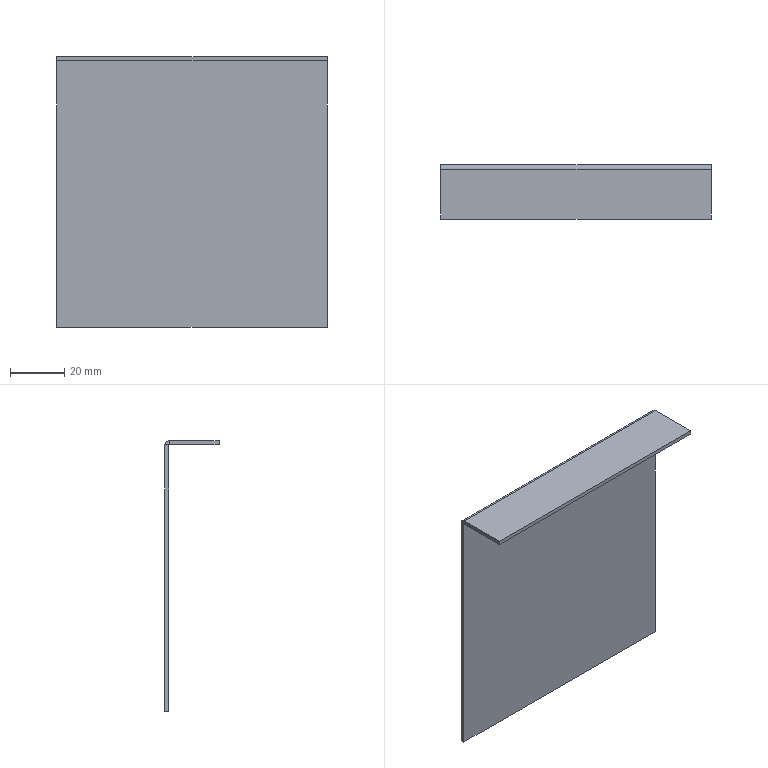Component | SolidWorks | WeldmentDrawing-1_CircuitBreakerBracket-1 | 1 solid | 14 faces | box 100 x 20 x 100 mm | volume 17720 mm3 | plane 12 | cylinder 2 | commonest cylinder face diameters 3.2 x1 0.2 x1
STEP:
#1=COLOUR_RGB('',0.7922,0.8196,0.9333);
#2=FILL_AREA_STYLE_COLOUR('',#1);
#3=FILL_AREA_STYLE('',(#2));
#4=SURFACE_STYLE_FILL_AREA(#3);
#5=SURFACE_SIDE_STYLE('',(#4));
#6=SURFACE_STYLE_USAGE(.BOTH.,#5);
#7=PRESENTATION_STYLE_ASSIGNMENT((#6));
#8=CARTESIAN_POINT('',(1.698,-7.825,-6.929));
#9=VERTEX_POINT('',#8);
#10=CARTESIAN_POINT('',(1.698,-7.825,-3.055));
#11=VERTEX_POINT('',#10);
#12=CARTESIAN_POINT('',(1.698,-7.825,-6.929));
#13=DIRECTION('',(-0.,-0.,1.));
#14=VECTOR('',#13,39.37);
#15=LINE('',#12,#14);
#16=EDGE_CURVE('',#9,#11,#15,.T.);
#17=ORIENTED_EDGE('',*,*,#16,.T.);
#18=CARTESIAN_POINT('',(1.698,-7.766,-3.055));
#19=VERTEX_POINT('',#18);
#20=CARTESIAN_POINT('',(1.698,-7.825,-3.055));
#21=DIRECTION('',(0.,1.,0.));
#22=VECTOR('',#21,39.37);
#23=LINE('',#20,#22);
#24=EDGE_CURVE('',#11,#19,#23,.T.);
#25=ORIENTED_EDGE('',*,*,#24,.T.);
#26=CARTESIAN_POINT('',(1.698,-7.766,-6.929));
#27=VERTEX_POINT('',#26);
#28=CARTESIAN_POINT('',(1.698,-7.766,-6.929));
#29=DIRECTION('',(-0.,-0.,1.));
#30=VECTOR('',#29,39.37);
#31=LINE('',#28,#30);
#32=EDGE_CURVE('',#27,#19,#31,.T.);
#33=ORIENTED_EDGE('',*,*,#32,.F.);
#34=CARTESIAN_POINT('',(1.698,-7.825,-6.929));
#35=DIRECTION('',(0.,1.,0.));
#36=VECTOR('',#35,39.37);
#37=LINE('',#34,#36);
#38=EDGE_CURVE('',#9,#27,#37,.T.);
#39=ORIENTED_EDGE('',*,*,#38,.F.);
#40=EDGE_LOOP('',(#17,#25,#33,#39));
#41=FACE_OUTER_BOUND('',#40,.T.);
#42=CARTESIAN_POINT('',(1.698,-7.825,-6.929));
#43=DIRECTION('',(-1.,-0.,-0.));
#44=DIRECTION('',(-0.,-0.,1.));
#45=AXIS2_PLACEMENT_3D('',#42,#43,#44);
#46=PLANE('',#45);
#47=ADVANCED_FACE('',(#41),#46,.T.);
#48=CARTESIAN_POINT('',(5.635,-7.825,-3.055));
#49=VERTEX_POINT('',#48);
#50=CARTESIAN_POINT('',(5.635,-7.825,-6.929));
#51=VERTEX_POINT('',#50);
#52=CARTESIAN_POINT('',(5.635,-7.825,-6.929));
#53=DIRECTION('',(0.,0.,-1.));
#54=VECTOR('',#53,39.37);
#55=LINE('',#52,#54);
#56=EDGE_CURVE('',#49,#51,#55,.T.);
#57=ORIENTED_EDGE('',*,*,#56,.F.);
#58=CARTESIAN_POINT('',(1.698,-7.825,-3.055));
#59=DIRECTION('',(1.,0.,0.));
#60=VECTOR('',#59,39.37);
#61=LINE('',#58,#60);
#62=EDGE_CURVE('',#11,#49,#61,.T.);
#63=ORIENTED_EDGE('',*,*,#62,.F.);
#64=ORIENTED_EDGE('',*,*,#16,.F.);
#65=CARTESIAN_POINT('',(5.635,-7.825,-6.929));
#66=DIRECTION('',(-1.,0.,-0.));
#67=VECTOR('',#66,39.37);
#68=LINE('',#65,#67);
#69=EDGE_CURVE('',#51,#9,#68,.T.);
#70=ORIENTED_EDGE('',*,*,#69,.F.);
#71=EDGE_LOOP('',(#57,#63,#64,#70));
#72=FACE_OUTER_BOUND('',#71,.T.);
#73=CARTESIAN_POINT('',(3.673,-7.825,-5.041));
#74=DIRECTION('',(-0.,-1.,-0.));
#75=DIRECTION('',(-0.,-0.,1.));
#76=AXIS2_PLACEMENT_3D('',#73,#74,#75);
#77=PLANE('',#76);
#78=ADVANCED_FACE('',(#72),#77,.T.);
#79=CARTESIAN_POINT('',(5.635,-7.766,-3.055));
#80=VERTEX_POINT('',#79);
#81=CARTESIAN_POINT('',(1.698,-7.766,-3.055));
#82=DIRECTION('',(1.,0.,0.));
#83=VECTOR('',#82,39.37);
#84=LINE('',#81,#83);
#85=EDGE_CURVE('',#19,#80,#84,.T.);
#86=ORIENTED_EDGE('',*,*,#85,.T.);
#87=CARTESIAN_POINT('',(5.635,-7.766,-6.929));
#88=VERTEX_POINT('',#87);
#89=CARTESIAN_POINT('',(5.635,-7.766,-6.929));
#90=DIRECTION('',(0.,0.,-1.));
#91=VECTOR('',#90,39.37);
#92=LINE('',#89,#91);
#93=EDGE_CURVE('',#80,#88,#92,.T.);
#94=ORIENTED_EDGE('',*,*,#93,.T.);
#95=CARTESIAN_POINT('',(5.635,-7.766,-6.929));
#96=DIRECTION('',(-1.,0.,-0.));
#97=VECTOR('',#96,39.37);
#98=LINE('',#95,#97);
#99=EDGE_CURVE('',#88,#27,#98,.T.);
#100=ORIENTED_EDGE('',*,*,#99,.T.);
#101=ORIENTED_EDGE('',*,*,#32,.T.);
#102=EDGE_LOOP('',(#86,#94,#100,#101));
#103=FACE_OUTER_BOUND('',#102,.T.);
#104=CARTESIAN_POINT('',(3.673,-7.766,-5.041));
#105=DIRECTION('',(-0.,-1.,-0.));
#106=DIRECTION('',(-0.,-0.,1.));
#107=AXIS2_PLACEMENT_3D('',#104,#105,#106);
#108=PLANE('',#107);
#109=ADVANCED_FACE('',(#103),#108,.F.);
#110=CARTESIAN_POINT('',(5.635,-7.825,-3.055));
#111=DIRECTION('',(0.,1.,0.));
#112=VECTOR('',#111,39.37);
#113=LINE('',#110,#112);
#114=EDGE_CURVE('',#49,#80,#113,.T.);
#115=ORIENTED_EDGE('',*,*,#114,.F.);
#116=ORIENTED_EDGE('',*,*,#56,.T.);
#117=CARTESIAN_POINT('',(5.635,-7.825,-6.929));
#118=DIRECTION('',(0.,1.,0.));
#119=VECTOR('',#118,39.37);
#120=LINE('',#117,#119);
#121=EDGE_CURVE('',#51,#88,#120,.T.);
#122=ORIENTED_EDGE('',*,*,#121,.T.);
#123=ORIENTED_EDGE('',*,*,#93,.F.);
#124=EDGE_LOOP('',(#115,#116,#122,#123));
#125=FACE_OUTER_BOUND('',#124,.T.);
#126=CARTESIAN_POINT('',(5.635,-7.825,-6.929));
#127=DIRECTION('',(1.,0.,0.));
#128=DIRECTION('',(0.,0.,-1.));
#129=AXIS2_PLACEMENT_3D('',#126,#127,#128);
#130=PLANE('',#129);
#131=ADVANCED_FACE('',(#125),#130,.T.);
#132=ORIENTED_EDGE('',*,*,#99,.F.);
#133=ORIENTED_EDGE('',*,*,#121,.F.);
#134=ORIENTED_EDGE('',*,*,#69,.T.);
#135=ORIENTED_EDGE('',*,*,#38,.T.);
#136=EDGE_LOOP('',(#132,#133,#134,#135));
#137=FACE_OUTER_BOUND('',#136,.T.);
#138=CARTESIAN_POINT('',(5.635,-7.825,-6.929));
#139=DIRECTION('',(0.,0.,-1.));
#140=DIRECTION('',(-1.,0.,-0.));
#141=AXIS2_PLACEMENT_3D('',#138,#139,#140);
#142=PLANE('',#141);
#143=ADVANCED_FACE('',(#137),#142,.T.);
#144=CARTESIAN_POINT('',(5.635,-7.829,-3.051));
#145=VERTEX_POINT('',#144);
#146=CARTESIAN_POINT('',(5.635,-7.829,-2.992));
#147=VERTEX_POINT('',#146);
#148=CARTESIAN_POINT('',(5.635,-7.829,-2.992));
#149=DIRECTION('',(-0.,-0.,1.));
#150=VECTOR('',#149,39.37);
#151=LINE('',#148,#150);
#152=EDGE_CURVE('',#145,#147,#151,.T.);
#153=ORIENTED_EDGE('',*,*,#152,.F.);
#154=CARTESIAN_POINT('',(5.635,-7.829,-3.055));
#155=DIRECTION('',(1.,0.,0.));
#156=DIRECTION('',(0.,0.,1.));
#157=AXIS2_PLACEMENT_3D('',#154,#155,#156);
#158=CIRCLE('',#157,0.003937);
#159=EDGE_CURVE('',#49,#145,#158,.T.);
#160=ORIENTED_EDGE('',*,*,#159,.F.);
#161=ORIENTED_EDGE('',*,*,#114,.T.);
#162=CARTESIAN_POINT('',(5.635,-7.829,-3.055));
#163=DIRECTION('',(1.,0.,0.));
#164=DIRECTION('',(0.,0.,1.));
#165=AXIS2_PLACEMENT_3D('',#162,#163,#164);
#166=CIRCLE('',#165,0.06299);
#167=EDGE_CURVE('',#80,#147,#166,.T.);
#168=ORIENTED_EDGE('',*,*,#167,.T.);
#169=EDGE_LOOP('',(#153,#160,#161,#168));
#170=FACE_OUTER_BOUND('',#169,.T.);
#171=CARTESIAN_POINT('',(5.635,-7.829,-3.055));
#172=DIRECTION('',(1.,0.,0.));
#173=DIRECTION('',(0.,0.,-1.));
#174=AXIS2_PLACEMENT_3D('',#171,#172,#173);
#175=PLANE('',#174);
#176=ADVANCED_FACE('',(#170),#175,.T.);
#177=CARTESIAN_POINT('',(1.698,-7.829,-3.051));
#178=VERTEX_POINT('',#177);
#179=CARTESIAN_POINT('',(1.698,-7.829,-3.055));
#180=DIRECTION('',(-1.,0.,-0.));
#181=DIRECTION('',(0.,0.,1.));
#182=AXIS2_PLACEMENT_3D('',#179,#180,#181);
#183=CIRCLE('',#182,0.003937);
#184=EDGE_CURVE('',#178,#11,#183,.T.);
#185=ORIENTED_EDGE('',*,*,#184,.F.);
#186=CARTESIAN_POINT('',(1.698,-7.829,-2.992));
#187=VERTEX_POINT('',#186);
#188=CARTESIAN_POINT('',(1.698,-7.829,-3.051));
#189=DIRECTION('',(-0.,-0.,1.));
#190=VECTOR('',#189,39.37);
#191=LINE('',#188,#190);
#192=EDGE_CURVE('',#178,#187,#191,.T.);
#193=ORIENTED_EDGE('',*,*,#192,.T.);
#194=CARTESIAN_POINT('',(1.698,-7.829,-3.055));
#195=DIRECTION('',(-1.,0.,-0.));
#196=DIRECTION('',(-0.,-0.,1.));
#197=AXIS2_PLACEMENT_3D('',#194,#195,#196);
#198=CIRCLE('',#197,0.06299);
#199=EDGE_CURVE('',#187,#19,#198,.T.);
#200=ORIENTED_EDGE('',*,*,#199,.T.);
#201=ORIENTED_EDGE('',*,*,#24,.F.);
#202=EDGE_LOOP('',(#185,#193,#200,#201));
#203=FACE_OUTER_BOUND('',#202,.T.);
#204=CARTESIAN_POINT('',(1.698,-7.829,-3.055));
#205=DIRECTION('',(1.,0.,0.));
#206=DIRECTION('',(0.,0.,-1.));
#207=AXIS2_PLACEMENT_3D('',#204,#205,#206);
#208=PLANE('',#207);
#209=ADVANCED_FACE('',(#203),#208,.F.);
#210=ORIENTED_EDGE('',*,*,#85,.F.);
#211=ORIENTED_EDGE('',*,*,#199,.F.);
#212=CARTESIAN_POINT('',(3.673,-7.829,-2.992));
#213=DIRECTION('',(-1.,0.,-0.));
#214=VECTOR('',#213,39.37);
#215=LINE('',#212,#214);
#216=EDGE_CURVE('',#147,#187,#215,.T.);
#217=ORIENTED_EDGE('',*,*,#216,.F.);
#218=ORIENTED_EDGE('',*,*,#167,.F.);
#219=EDGE_LOOP('',(#210,#211,#217,#218));
#220=FACE_OUTER_BOUND('',#219,.T.);
#221=CARTESIAN_POINT('',(1.698,-7.829,-3.055));
#222=DIRECTION('',(-1.,0.,-0.));
#223=DIRECTION('',(-0.,0.,1.));
#224=AXIS2_PLACEMENT_3D('',#221,#222,#223);
#225=CYLINDRICAL_SURFACE('',#224,0.06299);
#226=ADVANCED_FACE('',(#220),#225,.T.);
#227=ORIENTED_EDGE('',*,*,#62,.T.);
#228=ORIENTED_EDGE('',*,*,#159,.T.);
#229=CARTESIAN_POINT('',(5.635,-7.829,-3.051));
#230=DIRECTION('',(-1.,0.,-0.));
#231=VECTOR('',#230,39.37);
#232=LINE('',#229,#231);
#233=EDGE_CURVE('',#145,#178,#232,.T.);
#234=ORIENTED_EDGE('',*,*,#233,.T.);
#235=ORIENTED_EDGE('',*,*,#184,.T.);
#236=EDGE_LOOP('',(#227,#228,#234,#235));
#237=FACE_OUTER_BOUND('',#236,.T.);
#238=CARTESIAN_POINT('',(1.698,-7.829,-3.055));
#239=DIRECTION('',(-1.,0.,-0.));
#240=DIRECTION('',(0.,0.,1.));
#241=AXIS2_PLACEMENT_3D('',#238,#239,#240);
#242=CYLINDRICAL_SURFACE('',#241,0.003937);
#243=ADVANCED_FACE('',(#237),#242,.F.);
#244=CARTESIAN_POINT('',(1.698,-8.553,-2.992));
#245=VERTEX_POINT('',#244);
#246=CARTESIAN_POINT('',(1.698,-7.825,-2.992));
#247=DIRECTION('',(0.,1.,0.));
#248=VECTOR('',#247,39.37);
#249=LINE('',#246,#248);
#250=EDGE_CURVE('',#245,#187,#249,.T.);
#251=ORIENTED_EDGE('',*,*,#250,.T.);
#252=ORIENTED_EDGE('',*,*,#192,.F.);
#253=CARTESIAN_POINT('',(1.698,-8.553,-3.051));
#254=VERTEX_POINT('',#253);
#255=CARTESIAN_POINT('',(1.698,-7.766,-3.051));
#256=DIRECTION('',(0.,1.,0.));
#257=VECTOR('',#256,39.37);
#258=LINE('',#255,#257);
#259=EDGE_CURVE('',#254,#178,#258,.T.);
#260=ORIENTED_EDGE('',*,*,#259,.F.);
#261=CARTESIAN_POINT('',(1.698,-8.553,-2.992));
#262=DIRECTION('',(0.,0.,-1.));
#263=VECTOR('',#262,39.37);
#264=LINE('',#261,#263);
#265=EDGE_CURVE('',#245,#254,#264,.T.);
#266=ORIENTED_EDGE('',*,*,#265,.F.);
#267=EDGE_LOOP('',(#251,#252,#260,#266));
#268=FACE_OUTER_BOUND('',#267,.T.);
#269=CARTESIAN_POINT('',(1.698,-7.825,-2.992));
#270=DIRECTION('',(-1.,-0.,-0.));
#271=DIRECTION('',(-0.,-0.,1.));
#272=AXIS2_PLACEMENT_3D('',#269,#270,#271);
#273=PLANE('',#272);
#274=ADVANCED_FACE('',(#268),#273,.T.);
#275=CARTESIAN_POINT('',(5.635,-8.553,-3.051));
#276=VERTEX_POINT('',#275);
#277=CARTESIAN_POINT('',(5.635,-7.766,-3.051));
#278=DIRECTION('',(-0.,-1.,-0.));
#279=VECTOR('',#278,39.37);
#280=LINE('',#277,#279);
#281=EDGE_CURVE('',#145,#276,#280,.T.);
#282=ORIENTED_EDGE('',*,*,#281,.F.);
#283=ORIENTED_EDGE('',*,*,#152,.T.);
#284=CARTESIAN_POINT('',(5.635,-8.553,-2.992));
#285=VERTEX_POINT('',#284);
#286=CARTESIAN_POINT('',(5.635,-8.553,-2.992));
#287=DIRECTION('',(-0.,-1.,-0.));
#288=VECTOR('',#287,39.37);
#289=LINE('',#286,#288);
#290=EDGE_CURVE('',#147,#285,#289,.T.);
#291=ORIENTED_EDGE('',*,*,#290,.T.);
#292=CARTESIAN_POINT('',(5.635,-8.553,-2.992));
#293=DIRECTION('',(0.,0.,-1.));
#294=VECTOR('',#293,39.37);
#295=LINE('',#292,#294);
#296=EDGE_CURVE('',#285,#276,#295,.T.);
#297=ORIENTED_EDGE('',*,*,#296,.T.);
#298=EDGE_LOOP('',(#282,#283,#291,#297));
#299=FACE_OUTER_BOUND('',#298,.T.);
#300=CARTESIAN_POINT('',(5.635,-8.553,-2.992));
#301=DIRECTION('',(1.,0.,0.));
#302=DIRECTION('',(0.,0.,-1.));
#303=AXIS2_PLACEMENT_3D('',#300,#301,#302);
#304=PLANE('',#303);
#305=ADVANCED_FACE('',(#299),#304,.T.);
#306=ORIENTED_EDGE('',*,*,#290,.F.);
#307=ORIENTED_EDGE('',*,*,#216,.T.);
#308=ORIENTED_EDGE('',*,*,#250,.F.);
#309=CARTESIAN_POINT('',(1.698,-8.553,-2.992));
#310=DIRECTION('',(-1.,0.,-0.));
#311=VECTOR('',#310,39.37);
#312=LINE('',#309,#311);
#313=EDGE_CURVE('',#285,#245,#312,.T.);
#314=ORIENTED_EDGE('',*,*,#313,.F.);
#315=EDGE_LOOP('',(#306,#307,#308,#314));
#316=FACE_OUTER_BOUND('',#315,.T.);
#317=CARTESIAN_POINT('',(3.673,-7.766,-2.992));
#318=DIRECTION('',(-0.,-0.,1.));
#319=DIRECTION('',(0.,1.,0.));
#320=AXIS2_PLACEMENT_3D('',#317,#318,#319);
#321=PLANE('',#320);
#322=ADVANCED_FACE('',(#316),#321,.T.);
#323=ORIENTED_EDGE('',*,*,#233,.F.);
#324=ORIENTED_EDGE('',*,*,#281,.T.);
#325=CARTESIAN_POINT('',(3.673,-8.553,-3.051));
#326=DIRECTION('',(-1.,0.,-0.));
#327=VECTOR('',#326,39.37);
#328=LINE('',#325,#327);
#329=EDGE_CURVE('',#276,#254,#328,.T.);
#330=ORIENTED_EDGE('',*,*,#329,.T.);
#331=ORIENTED_EDGE('',*,*,#259,.T.);
#332=EDGE_LOOP('',(#323,#324,#330,#331));
#333=FACE_OUTER_BOUND('',#332,.T.);
#334=CARTESIAN_POINT('',(3.673,-7.766,-3.051));
#335=DIRECTION('',(-0.,-0.,1.));
#336=DIRECTION('',(0.,1.,0.));
#337=AXIS2_PLACEMENT_3D('',#334,#335,#336);
#338=PLANE('',#337);
#339=ADVANCED_FACE('',(#333),#338,.F.);
#340=ORIENTED_EDGE('',*,*,#329,.F.);
#341=ORIENTED_EDGE('',*,*,#296,.F.);
#342=ORIENTED_EDGE('',*,*,#313,.T.);
#343=ORIENTED_EDGE('',*,*,#265,.T.);
#344=EDGE_LOOP('',(#340,#341,#342,#343));
#345=FACE_OUTER_BOUND('',#344,.T.);
#346=CARTESIAN_POINT('',(1.698,-8.553,-2.992));
#347=DIRECTION('',(-0.,-1.,-0.));
#348=DIRECTION('',(-0.,-0.,1.));
#349=AXIS2_PLACEMENT_3D('',#346,#347,#348);
#350=PLANE('',#349);
#351=ADVANCED_FACE('',(#345),#350,.T.);
#352=CLOSED_SHELL('',(#47,#78,#109,#131,#143,#176,#209,#226,#243,#274,#305,#322,#339,#351));
#353=MANIFOLD_SOLID_BREP('',#352);
#354=STYLED_ITEM('',(#7),#353);
#355=PRESENTATION_LAYER_ASSIGNMENT('','',(#354));
#356=CARTESIAN_POINT('',(0.,0.,0.));
#357=DIRECTION('',(0.,0.,1.));
#358=DIRECTION('',(1.,0.,0.));
#359=AXIS2_PLACEMENT_3D('',#356,#357,#358);
#360=(LENGTH_UNIT()NAMED_UNIT(*)SI_UNIT($,.METRE.));
#361=LENGTH_MEASURE_WITH_UNIT(LENGTH_MEASURE(0.0254),#360);
#362=DIMENSIONAL_EXPONENTS(1.,0.,0.,0.,0.,0.,0.);
#363=(CONVERSION_BASED_UNIT('',#361)LENGTH_UNIT()NAMED_UNIT(#362));
#364=UNCERTAINTY_MEASURE_WITH_UNIT(LENGTH_MEASURE(0.00001),#363,'','');
#365=(NAMED_UNIT(*)PLANE_ANGLE_UNIT()SI_UNIT($,.RADIAN.));
#366=(NAMED_UNIT(*)SI_UNIT($,.STERADIAN.)SOLID_ANGLE_UNIT());
#367=(GEOMETRIC_REPRESENTATION_CONTEXT(3)GLOBAL_UNCERTAINTY_ASSIGNED_CONTEXT((#364))GLOBAL_UNIT_ASSIGNED_CONTEXT((#363,#365,#366))REPRESENTATION_CONTEXT('',''));
#368=ADVANCED_BREP_SHAPE_REPRESENTATION('',(#353,#359),#367);
#369=(LENGTH_UNIT()NAMED_UNIT(*)SI_UNIT($,.METRE.));
#370=LENGTH_MEASURE_WITH_UNIT(LENGTH_MEASURE(0.0254),#369);
#371=DIMENSIONAL_EXPONENTS(1.,0.,0.,0.,0.,0.,0.);
#372=(CONVERSION_BASED_UNIT('',#370)LENGTH_UNIT()NAMED_UNIT(#371));
#373=UNCERTAINTY_MEASURE_WITH_UNIT(LENGTH_MEASURE(0.00001),#372,'','');
#374=(NAMED_UNIT(*)PLANE_ANGLE_UNIT()SI_UNIT($,.RADIAN.));
#375=(NAMED_UNIT(*)SI_UNIT($,.STERADIAN.)SOLID_ANGLE_UNIT());
#376=(GEOMETRIC_REPRESENTATION_CONTEXT(3)GLOBAL_UNCERTAINTY_ASSIGNED_CONTEXT((#373))GLOBAL_UNIT_ASSIGNED_CONTEXT((#372,#374,#375))REPRESENTATION_CONTEXT('',''));
#377=MECHANICAL_DESIGN_GEOMETRIC_PRESENTATION_REPRESENTATION('',(#354),#376);